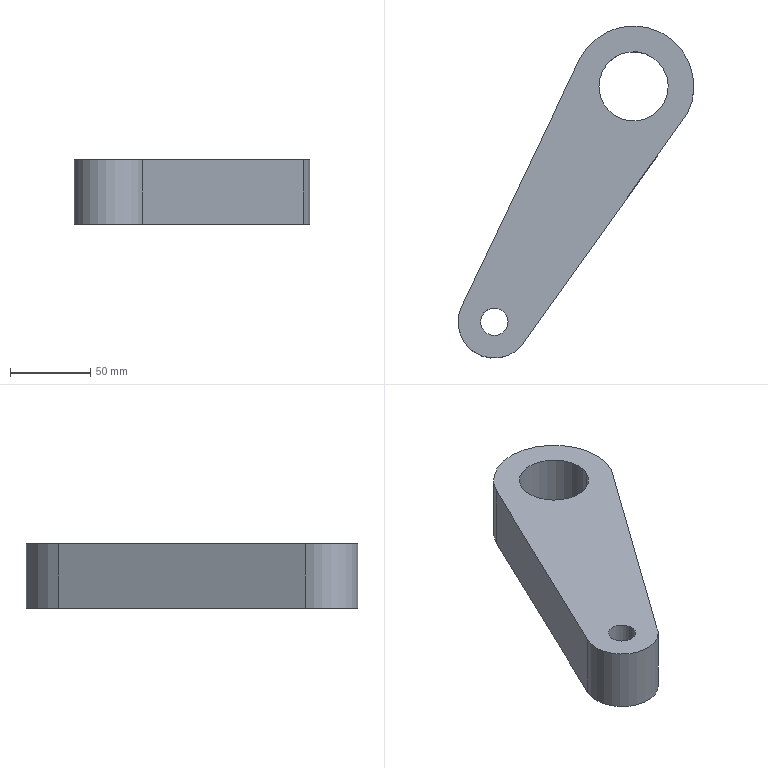Component | SolidWorks | ConnectingRod1-1 | 1 solid | 10 faces | box 146.49 x 206.35 x 40 mm | volume 460221 mm3 | cylinder 6 | plane 4 | commonest cylinder face diameters 43 x2 17 x2 45 x1 75 x1 | material 45
build123d program:
from build123d import *

# Parameters (mm, degrees)
SKETCH1_R           = 8.5
SKETCH1_R_2         = 21.5
BOSS_EXTRUDE1_DEPTH = 20


with BuildPart() as part:
    # Sketch1 → Boss-Extrude1 (new, symmetric)
    with BuildSketch(Plane.XY):
        with BuildLine():
            Line((1425.717, -496.069), (1427.372, -485.05))
            ThreePointArc((1427.372, -485.05), (1389.872, -447.55), (1352.372, -485.05))
            Line((1352.372, -485.05), (1352.425, -487.042))
            Line((1352.425, -487.042), (1356.881, -654.726))
            ThreePointArc((1356.881, -654.726), (1379.381, -677.226), (1401.881, -654.726))
            Line((1401.881, -654.726), (1425.717, -496.069))
        make_face()
        with Locations((1379.381, -654.726)):
            Circle(SKETCH1_R, mode=Mode.SUBTRACT)
        with Locations((1389.872, -485.05)):
            Circle(SKETCH1_R_2, mode=Mode.SUBTRACT)
    extrude(amount=BOSS_EXTRUDE1_DEPTH, both=True)


solid = part.part

# Placed as in the assembly
solid = solid.moved(Location((468.852, 496.589, -220), (0, 0, -27.045)))
STEP:
#1=COLOUR_RGB('',0.7922,0.8196,0.9333);
#2=FILL_AREA_STYLE_COLOUR('',#1);
#3=FILL_AREA_STYLE('',(#2));
#4=SURFACE_STYLE_FILL_AREA(#3);
#5=SURFACE_SIDE_STYLE('',(#4));
#6=SURFACE_STYLE_USAGE(.BOTH.,#5);
#7=PRESENTATION_STYLE_ASSIGNMENT((#6));
#8=CARTESIAN_POINT('',(57.758,-21.953,-7.874));
#9=VERTEX_POINT('',#8);
#10=CARTESIAN_POINT('',(59.266,-22.723,-7.874));
#11=VERTEX_POINT('',#10);
#12=CARTESIAN_POINT('',(58.512,-22.338,-7.874));
#13=DIRECTION('',(-0.,-0.,1.));
#14=DIRECTION('',(0.8907,-0.4547,0.));
#15=AXIS2_PLACEMENT_3D('',#12,#13,#14);
#16=CIRCLE('',#15,0.8465);
#17=EDGE_CURVE('',#9,#11,#16,.T.);
#18=ORIENTED_EDGE('',*,*,#17,.T.);
#19=CARTESIAN_POINT('',(59.266,-22.723,-9.449));
#20=VERTEX_POINT('',#19);
#21=CARTESIAN_POINT('',(59.266,-22.723,-7.874));
#22=DIRECTION('',(0.,0.,-1.));
#23=VECTOR('',#22,39.37);
#24=LINE('',#21,#23);
#25=EDGE_CURVE('',#11,#20,#24,.T.);
#26=ORIENTED_EDGE('',*,*,#25,.T.);
#27=CARTESIAN_POINT('',(57.758,-21.953,-9.449));
#28=VERTEX_POINT('',#27);
#29=CARTESIAN_POINT('',(58.512,-22.338,-9.449));
#30=DIRECTION('',(-0.,-0.,1.));
#31=DIRECTION('',(0.8907,-0.4547,0.));
#32=AXIS2_PLACEMENT_3D('',#29,#30,#31);
#33=CIRCLE('',#32,0.8465);
#34=EDGE_CURVE('',#28,#20,#33,.T.);
#35=ORIENTED_EDGE('',*,*,#34,.F.);
#36=CARTESIAN_POINT('',(57.758,-21.953,-7.874));
#37=DIRECTION('',(0.,0.,-1.));
#38=VECTOR('',#37,39.37);
#39=LINE('',#36,#38);
#40=EDGE_CURVE('',#9,#28,#39,.T.);
#41=ORIENTED_EDGE('',*,*,#40,.F.);
#42=EDGE_LOOP('',(#18,#26,#35,#41));
#43=FACE_OUTER_BOUND('',#42,.T.);
#44=CARTESIAN_POINT('',(58.512,-22.338,-7.874));
#45=DIRECTION('',(0.,0.,-1.));
#46=DIRECTION('',(-0.8907,0.4547,0.));
#47=AXIS2_PLACEMENT_3D('',#44,#45,#46);
#48=CYLINDRICAL_SURFACE('',#47,0.8465);
#49=ADVANCED_FACE('',(#43),#48,.F.);
#50=CARTESIAN_POINT('',(54.809,-27.947,-7.874));
#51=VERTEX_POINT('',#50);
#52=CARTESIAN_POINT('',(55.405,-28.252,-7.874));
#53=VERTEX_POINT('',#52);
#54=CARTESIAN_POINT('',(55.107,-28.1,-7.874));
#55=DIRECTION('',(-0.,-0.,1.));
#56=DIRECTION('',(0.8907,-0.4547,0.));
#57=AXIS2_PLACEMENT_3D('',#54,#55,#56);
#58=CIRCLE('',#57,0.3346);
#59=EDGE_CURVE('',#51,#53,#58,.T.);
#60=ORIENTED_EDGE('',*,*,#59,.T.);
#61=CARTESIAN_POINT('',(55.405,-28.252,-9.449));
#62=VERTEX_POINT('',#61);
#63=CARTESIAN_POINT('',(55.405,-28.252,-7.874));
#64=DIRECTION('',(0.,0.,-1.));
#65=VECTOR('',#64,39.37);
#66=LINE('',#63,#65);
#67=EDGE_CURVE('',#53,#62,#66,.T.);
#68=ORIENTED_EDGE('',*,*,#67,.T.);
#69=CARTESIAN_POINT('',(54.809,-27.947,-9.449));
#70=VERTEX_POINT('',#69);
#71=CARTESIAN_POINT('',(55.107,-28.1,-9.449));
#72=DIRECTION('',(-0.,-0.,1.));
#73=DIRECTION('',(0.8907,-0.4547,0.));
#74=AXIS2_PLACEMENT_3D('',#71,#72,#73);
#75=CIRCLE('',#74,0.3346);
#76=EDGE_CURVE('',#70,#62,#75,.T.);
#77=ORIENTED_EDGE('',*,*,#76,.F.);
#78=CARTESIAN_POINT('',(54.809,-27.947,-7.874));
#79=DIRECTION('',(0.,0.,-1.));
#80=VECTOR('',#79,39.37);
#81=LINE('',#78,#80);
#82=EDGE_CURVE('',#51,#70,#81,.T.);
#83=ORIENTED_EDGE('',*,*,#82,.F.);
#84=EDGE_LOOP('',(#60,#68,#77,#83));
#85=FACE_OUTER_BOUND('',#84,.T.);
#86=CARTESIAN_POINT('',(55.107,-28.1,-7.874));
#87=DIRECTION('',(0.,0.,-1.));
#88=DIRECTION('',(-0.8907,0.4547,0.));
#89=AXIS2_PLACEMENT_3D('',#86,#87,#88);
#90=CYLINDRICAL_SURFACE('',#89,0.3346);
#91=ADVANCED_FACE('',(#85),#90,.F.);
#92=CARTESIAN_POINT('',(57.197,-21.666,-9.449));
#93=VERTEX_POINT('',#92);
#94=CARTESIAN_POINT('',(54.318,-27.697,-9.449));
#95=VERTEX_POINT('',#94);
#96=CARTESIAN_POINT('',(66.031,-3.163,-9.449));
#97=DIRECTION('',(-0.4309,-0.9024,-0.));
#98=VECTOR('',#97,39.37);
#99=LINE('',#96,#98);
#100=EDGE_CURVE('',#93,#95,#99,.T.);
#101=ORIENTED_EDGE('',*,*,#100,.T.);
#102=CARTESIAN_POINT('',(54.318,-27.697,-7.874));
#103=VERTEX_POINT('',#102);
#104=CARTESIAN_POINT('',(54.318,-27.697,-7.874));
#105=DIRECTION('',(0.,0.,-1.));
#106=VECTOR('',#105,39.37);
#107=LINE('',#104,#106);
#108=EDGE_CURVE('',#103,#95,#107,.T.);
#109=ORIENTED_EDGE('',*,*,#108,.F.);
#110=CARTESIAN_POINT('',(57.197,-21.666,-7.874));
#111=VERTEX_POINT('',#110);
#112=CARTESIAN_POINT('',(66.031,-3.163,-7.874));
#113=DIRECTION('',(-0.4309,-0.9024,-0.));
#114=VECTOR('',#113,39.37);
#115=LINE('',#112,#114);
#116=EDGE_CURVE('',#111,#103,#115,.T.);
#117=ORIENTED_EDGE('',*,*,#116,.F.);
#118=CARTESIAN_POINT('',(57.197,-21.666,-7.874));
#119=DIRECTION('',(0.,0.,-1.));
#120=VECTOR('',#119,39.37);
#121=LINE('',#118,#120);
#122=EDGE_CURVE('',#111,#93,#121,.T.);
#123=ORIENTED_EDGE('',*,*,#122,.T.);
#124=EDGE_LOOP('',(#101,#109,#117,#123));
#125=FACE_OUTER_BOUND('',#124,.T.);
#126=CARTESIAN_POINT('',(66.031,-3.163,-7.874));
#127=DIRECTION('',(0.9024,-0.4309,0.));
#128=DIRECTION('',(0.4309,0.9024,0.));
#129=AXIS2_PLACEMENT_3D('',#126,#127,#128);
#130=PLANE('',#129);
#131=ADVANCED_FACE('',(#125),#130,.F.);
#132=CARTESIAN_POINT('',(55.896,-28.502,-9.449));
#133=VERTEX_POINT('',#132);
#134=CARTESIAN_POINT('',(55.107,-28.1,-9.449));
#135=DIRECTION('',(-0.,-0.,1.));
#136=DIRECTION('',(0.8907,-0.4547,0.));
#137=AXIS2_PLACEMENT_3D('',#134,#135,#136);
#138=CIRCLE('',#137,0.8858);
#139=EDGE_CURVE('',#95,#133,#138,.T.);
#140=ORIENTED_EDGE('',*,*,#139,.T.);
#141=CARTESIAN_POINT('',(55.896,-28.502,-7.874));
#142=VERTEX_POINT('',#141);
#143=CARTESIAN_POINT('',(55.896,-28.502,-7.874));
#144=DIRECTION('',(0.,0.,-1.));
#145=VECTOR('',#144,39.37);
#146=LINE('',#143,#145);
#147=EDGE_CURVE('',#142,#133,#146,.T.);
#148=ORIENTED_EDGE('',*,*,#147,.F.);
#149=CARTESIAN_POINT('',(55.107,-28.1,-7.874));
#150=DIRECTION('',(-0.,-0.,1.));
#151=DIRECTION('',(0.8907,-0.4547,0.));
#152=AXIS2_PLACEMENT_3D('',#149,#150,#151);
#153=CIRCLE('',#152,0.8858);
#154=EDGE_CURVE('',#103,#142,#153,.T.);
#155=ORIENTED_EDGE('',*,*,#154,.F.);
#156=ORIENTED_EDGE('',*,*,#108,.T.);
#157=EDGE_LOOP('',(#140,#148,#155,#156));
#158=FACE_OUTER_BOUND('',#157,.T.);
#159=CARTESIAN_POINT('',(55.107,-28.1,-7.874));
#160=DIRECTION('',(0.,0.,-1.));
#161=DIRECTION('',(-0.8907,0.4547,0.));
#162=AXIS2_PLACEMENT_3D('',#159,#160,#161);
#163=CYLINDRICAL_SURFACE('',#162,0.8858);
#164=ADVANCED_FACE('',(#158),#163,.T.);
#165=CARTESIAN_POINT('',(59.827,-23.009,-9.449));
#166=VERTEX_POINT('',#165);
#167=CARTESIAN_POINT('',(65.958,-14.441,-9.449));
#168=DIRECTION('',(-0.582,-0.8132,-0.));
#169=VECTOR('',#168,39.37);
#170=LINE('',#167,#169);
#171=EDGE_CURVE('',#166,#133,#170,.T.);
#172=ORIENTED_EDGE('',*,*,#171,.F.);
#173=CARTESIAN_POINT('',(59.827,-23.009,-7.874));
#174=VERTEX_POINT('',#173);
#175=CARTESIAN_POINT('',(59.827,-23.009,-7.874));
#176=DIRECTION('',(0.,0.,-1.));
#177=VECTOR('',#176,39.37);
#178=LINE('',#175,#177);
#179=EDGE_CURVE('',#174,#166,#178,.T.);
#180=ORIENTED_EDGE('',*,*,#179,.F.);
#181=CARTESIAN_POINT('',(65.958,-14.441,-7.874));
#182=DIRECTION('',(-0.582,-0.8132,-0.));
#183=VECTOR('',#182,39.37);
#184=LINE('',#181,#183);
#185=EDGE_CURVE('',#174,#142,#184,.T.);
#186=ORIENTED_EDGE('',*,*,#185,.T.);
#187=ORIENTED_EDGE('',*,*,#147,.T.);
#188=EDGE_LOOP('',(#172,#180,#186,#187));
#189=FACE_OUTER_BOUND('',#188,.T.);
#190=CARTESIAN_POINT('',(65.958,-14.441,-7.874));
#191=DIRECTION('',(0.8132,-0.582,0.));
#192=DIRECTION('',(0.582,0.8132,0.));
#193=AXIS2_PLACEMENT_3D('',#190,#191,#192);
#194=PLANE('',#193);
#195=ADVANCED_FACE('',(#189),#194,.T.);
#196=ORIENTED_EDGE('',*,*,#67,.F.);
#197=CARTESIAN_POINT('',(55.107,-28.1,-7.874));
#198=DIRECTION('',(-0.,-0.,1.));
#199=DIRECTION('',(0.8907,-0.4547,0.));
#200=AXIS2_PLACEMENT_3D('',#197,#198,#199);
#201=CIRCLE('',#200,0.3346);
#202=EDGE_CURVE('',#53,#51,#201,.T.);
#203=ORIENTED_EDGE('',*,*,#202,.T.);
#204=ORIENTED_EDGE('',*,*,#82,.T.);
#205=CARTESIAN_POINT('',(55.107,-28.1,-9.449));
#206=DIRECTION('',(-0.,-0.,1.));
#207=DIRECTION('',(0.8907,-0.4547,0.));
#208=AXIS2_PLACEMENT_3D('',#205,#206,#207);
#209=CIRCLE('',#208,0.3346);
#210=EDGE_CURVE('',#62,#70,#209,.T.);
#211=ORIENTED_EDGE('',*,*,#210,.F.);
#212=EDGE_LOOP('',(#196,#203,#204,#211));
#213=FACE_OUTER_BOUND('',#212,.T.);
#214=CARTESIAN_POINT('',(55.107,-28.1,-7.874));
#215=DIRECTION('',(0.,0.,-1.));
#216=DIRECTION('',(-0.8907,0.4547,0.));
#217=AXIS2_PLACEMENT_3D('',#214,#215,#216);
#218=CYLINDRICAL_SURFACE('',#217,0.3346);
#219=ADVANCED_FACE('',(#213),#218,.F.);
#220=ORIENTED_EDGE('',*,*,#25,.F.);
#221=CARTESIAN_POINT('',(58.512,-22.338,-7.874));
#222=DIRECTION('',(-0.,-0.,1.));
#223=DIRECTION('',(0.8907,-0.4547,0.));
#224=AXIS2_PLACEMENT_3D('',#221,#222,#223);
#225=CIRCLE('',#224,0.8465);
#226=EDGE_CURVE('',#11,#9,#225,.T.);
#227=ORIENTED_EDGE('',*,*,#226,.T.);
#228=ORIENTED_EDGE('',*,*,#40,.T.);
#229=CARTESIAN_POINT('',(58.512,-22.338,-9.449));
#230=DIRECTION('',(-0.,-0.,1.));
#231=DIRECTION('',(0.8907,-0.4547,0.));
#232=AXIS2_PLACEMENT_3D('',#229,#230,#231);
#233=CIRCLE('',#232,0.8465);
#234=EDGE_CURVE('',#20,#28,#233,.T.);
#235=ORIENTED_EDGE('',*,*,#234,.F.);
#236=EDGE_LOOP('',(#220,#227,#228,#235));
#237=FACE_OUTER_BOUND('',#236,.T.);
#238=CARTESIAN_POINT('',(58.512,-22.338,-7.874));
#239=DIRECTION('',(0.,0.,-1.));
#240=DIRECTION('',(-0.8907,0.4547,0.));
#241=AXIS2_PLACEMENT_3D('',#238,#239,#240);
#242=CYLINDRICAL_SURFACE('',#241,0.8465);
#243=ADVANCED_FACE('',(#237),#242,.F.);
#244=CARTESIAN_POINT('',(58.512,-22.338,-9.449));
#245=DIRECTION('',(-0.,-0.,1.));
#246=DIRECTION('',(0.8907,-0.4547,0.));
#247=AXIS2_PLACEMENT_3D('',#244,#245,#246);
#248=CIRCLE('',#247,1.476);
#249=EDGE_CURVE('',#166,#93,#248,.T.);
#250=ORIENTED_EDGE('',*,*,#249,.T.);
#251=ORIENTED_EDGE('',*,*,#122,.F.);
#252=CARTESIAN_POINT('',(58.512,-22.338,-7.874));
#253=DIRECTION('',(-0.,-0.,1.));
#254=DIRECTION('',(0.8907,-0.4547,0.));
#255=AXIS2_PLACEMENT_3D('',#252,#253,#254);
#256=CIRCLE('',#255,1.476);
#257=EDGE_CURVE('',#174,#111,#256,.T.);
#258=ORIENTED_EDGE('',*,*,#257,.F.);
#259=ORIENTED_EDGE('',*,*,#179,.T.);
#260=EDGE_LOOP('',(#250,#251,#258,#259));
#261=FACE_OUTER_BOUND('',#260,.T.);
#262=CARTESIAN_POINT('',(58.512,-22.338,-7.874));
#263=DIRECTION('',(0.,0.,-1.));
#264=DIRECTION('',(-0.8907,0.4547,0.));
#265=AXIS2_PLACEMENT_3D('',#262,#263,#264);
#266=CYLINDRICAL_SURFACE('',#265,1.476);
#267=ADVANCED_FACE('',(#261),#266,.T.);
#268=ORIENTED_EDGE('',*,*,#17,.F.);
#269=ORIENTED_EDGE('',*,*,#226,.F.);
#270=EDGE_LOOP('',(#268,#269));
#271=FACE_BOUND('',#270,.T.);
#272=ORIENTED_EDGE('',*,*,#59,.F.);
#273=ORIENTED_EDGE('',*,*,#202,.F.);
#274=EDGE_LOOP('',(#272,#273));
#275=FACE_BOUND('',#274,.T.);
#276=ORIENTED_EDGE('',*,*,#116,.T.);
#277=ORIENTED_EDGE('',*,*,#154,.T.);
#278=ORIENTED_EDGE('',*,*,#185,.F.);
#279=ORIENTED_EDGE('',*,*,#257,.T.);
#280=EDGE_LOOP('',(#276,#277,#278,#279));
#281=FACE_OUTER_BOUND('',#280,.T.);
#282=CARTESIAN_POINT('',(18.459,19.551,-7.874));
#283=DIRECTION('',(-0.,-0.,1.));
#284=DIRECTION('',(0.8907,-0.4547,0.));
#285=AXIS2_PLACEMENT_3D('',#282,#283,#284);
#286=PLANE('',#285);
#287=ADVANCED_FACE('',(#271,#275,#281),#286,.T.);
#288=ORIENTED_EDGE('',*,*,#34,.T.);
#289=ORIENTED_EDGE('',*,*,#234,.T.);
#290=EDGE_LOOP('',(#288,#289));
#291=FACE_BOUND('',#290,.T.);
#292=ORIENTED_EDGE('',*,*,#76,.T.);
#293=ORIENTED_EDGE('',*,*,#210,.T.);
#294=EDGE_LOOP('',(#292,#293));
#295=FACE_BOUND('',#294,.T.);
#296=ORIENTED_EDGE('',*,*,#100,.F.);
#297=ORIENTED_EDGE('',*,*,#249,.F.);
#298=ORIENTED_EDGE('',*,*,#171,.T.);
#299=ORIENTED_EDGE('',*,*,#139,.F.);
#300=EDGE_LOOP('',(#296,#297,#298,#299));
#301=FACE_OUTER_BOUND('',#300,.T.);
#302=CARTESIAN_POINT('',(18.459,19.551,-9.449));
#303=DIRECTION('',(-0.,-0.,1.));
#304=DIRECTION('',(0.8907,-0.4547,0.));
#305=AXIS2_PLACEMENT_3D('',#302,#303,#304);
#306=PLANE('',#305);
#307=ADVANCED_FACE('',(#291,#295,#301),#306,.F.);
#308=CLOSED_SHELL('',(#49,#91,#131,#164,#195,#219,#243,#267,#287,#307));
#309=MANIFOLD_SOLID_BREP('',#308);
#310=STYLED_ITEM('',(#7),#309);
#311=(LENGTH_UNIT()NAMED_UNIT(*)SI_UNIT($,.METRE.));
#312=LENGTH_MEASURE_WITH_UNIT(LENGTH_MEASURE(0.0254),#311);
#313=DIMENSIONAL_EXPONENTS(1.,0.,0.,0.,0.,0.,0.);
#314=(CONVERSION_BASED_UNIT('',#312)LENGTH_UNIT()NAMED_UNIT(#313));
#315=UNCERTAINTY_MEASURE_WITH_UNIT(LENGTH_MEASURE(0.00001),#314,'','');
#316=(NAMED_UNIT(*)PLANE_ANGLE_UNIT()SI_UNIT($,.RADIAN.));
#317=(NAMED_UNIT(*)SI_UNIT($,.STERADIAN.)SOLID_ANGLE_UNIT());
#318=(GEOMETRIC_REPRESENTATION_CONTEXT(3)GLOBAL_UNCERTAINTY_ASSIGNED_CONTEXT((#315))GLOBAL_UNIT_ASSIGNED_CONTEXT((#314,#316,#317))REPRESENTATION_CONTEXT('',''));
#319=MECHANICAL_DESIGN_GEOMETRIC_PRESENTATION_REPRESENTATION('',(#310),#318);
#320=PRESENTATION_LAYER_ASSIGNMENT('','',(#310));
#321=CARTESIAN_POINT('',(0.,0.,0.));
#322=DIRECTION('',(0.,0.,1.));
#323=DIRECTION('',(1.,0.,0.));
#324=AXIS2_PLACEMENT_3D('',#321,#322,#323);
#325=(LENGTH_UNIT()NAMED_UNIT(*)SI_UNIT($,.METRE.));
#326=LENGTH_MEASURE_WITH_UNIT(LENGTH_MEASURE(0.0254),#325);
#327=DIMENSIONAL_EXPONENTS(1.,0.,0.,0.,0.,0.,0.);
#328=(CONVERSION_BASED_UNIT('',#326)LENGTH_UNIT()NAMED_UNIT(#327));
#329=UNCERTAINTY_MEASURE_WITH_UNIT(LENGTH_MEASURE(0.00001),#328,'','');
#330=(NAMED_UNIT(*)PLANE_ANGLE_UNIT()SI_UNIT($,.RADIAN.));
#331=(NAMED_UNIT(*)SI_UNIT($,.STERADIAN.)SOLID_ANGLE_UNIT());
#332=(GEOMETRIC_REPRESENTATION_CONTEXT(3)GLOBAL_UNCERTAINTY_ASSIGNED_CONTEXT((#329))GLOBAL_UNIT_ASSIGNED_CONTEXT((#328,#330,#331))REPRESENTATION_CONTEXT('',''));
#333=ADVANCED_BREP_SHAPE_REPRESENTATION('',(#309,#324),#332);